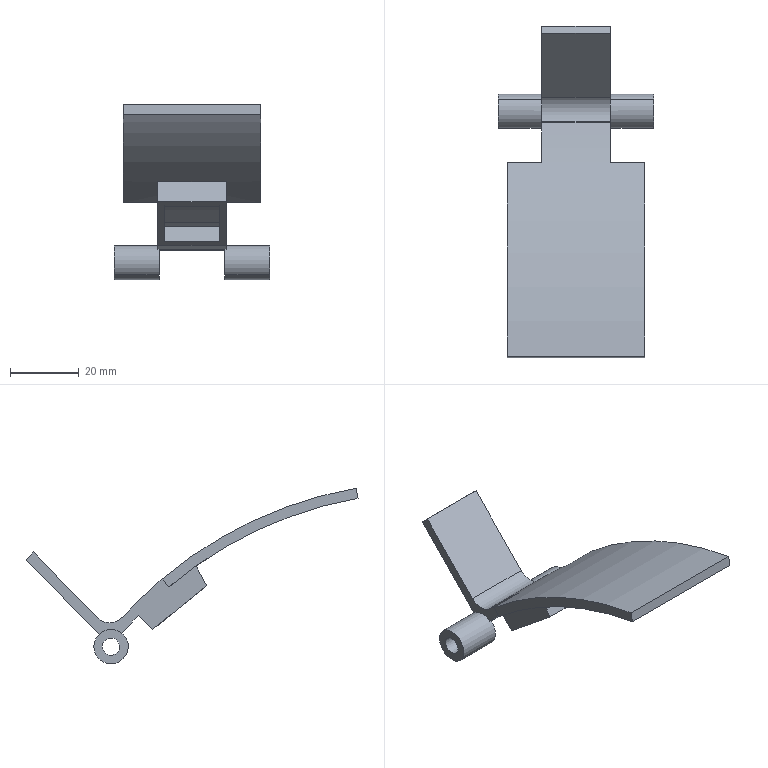Component | SolidWorks | SeedingAssemblyA-1_PressingPlate-1 | 1 solid | 37 faces | volume 13072 mm3 | plane 21 | cylinder 16 | commonest cylinder face diameters 10 x7 234 x4 5 x4 240 x1